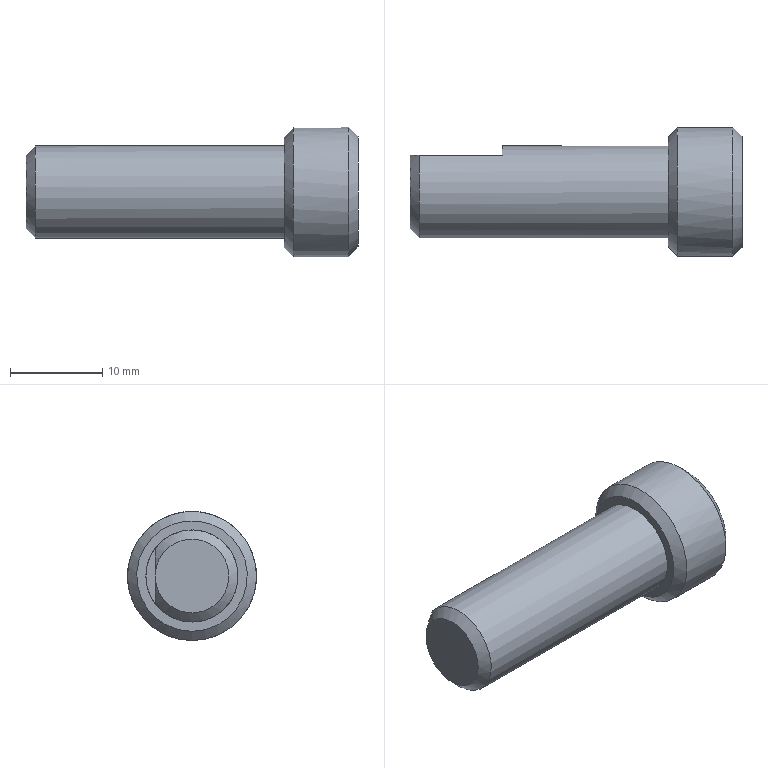Component | NX | 9_LEVER | 1 solid | 10 faces | box 36 x 14 x 14 mm | volume 3336 mm3 | plane 5 | cone 3 | cylinder 2 | commonest cylinder face diameters 10 x1 14 x1
STEP:
#1=CARTESIAN_POINT('',(0.,0.,0.));
#2=DIRECTION('',(0.,0.,1.));
#3=DIRECTION('',(1.,0.,0.));
#4=AXIS2_PLACEMENT_3D('',#1,#2,#3);
#5=CARTESIAN_POINT('',(14.,4.,75.));
#6=VERTEX_POINT('',#5);
#7=CARTESIAN_POINT('',(14.,-0.,75.));
#8=DIRECTION('',(-1.,0.,-0.));
#9=DIRECTION('',(0.,0.,-1.));
#10=AXIS2_PLACEMENT_3D('',#7,#8,#9);
#11=CIRCLE('',#10,4.);
#12=CARTESIAN_POINT('',(14.,-0.,75.));
#13=DIRECTION('',(1.,0.,0.));
#14=DIRECTION('',(0.,0.,-1.));
#15=AXIS2_PLACEMENT_3D('',#12,#13,#14);
#16=PLANE('',#15);
#17=CARTESIAN_POINT('',(4.,0.));
#18=CARTESIAN_POINT('',(4.,-6.928));
#19=CARTESIAN_POINT('',(-2.,-3.464));
#20=CARTESIAN_POINT('',(-8.,-0.));
#21=CARTESIAN_POINT('',(-2.,3.464));
#22=CARTESIAN_POINT('',(4.,6.928));
#23=CARTESIAN_POINT('',(4.,0.));
#24=(BOUNDED_CURVE()B_SPLINE_CURVE(2,(#17,#18,#19,#20,#21,#22,#23),.UNSPECIFIED.,.T.,.F.)B_SPLINE_CURVE_WITH_KNOTS((1,2,2,2,2,1),(-2.094,0.,2.094,4.189,6.283,8.378),.UNSPECIFIED.)CURVE()GEOMETRIC_REPRESENTATION_ITEM()RATIONAL_B_SPLINE_CURVE((1.,0.5,1.,0.5,1.,0.5,1.))REPRESENTATION_ITEM(''));
#25=(GEOMETRIC_REPRESENTATION_CONTEXT(2)PARAMETRIC_REPRESENTATION_CONTEXT()REPRESENTATION_CONTEXT('',''));
#26=DEFINITIONAL_REPRESENTATION('',(#24),#25);
#27=PCURVE('',#16,#26);
#28=CARTESIAN_POINT('',(15.,-0.,75.));
#29=DIRECTION('',(1.,0.,0.));
#30=DIRECTION('',(0.,0.,-1.));
#31=AXIS2_PLACEMENT_3D('',#28,#29,#30);
#32=CONICAL_SURFACE('',#31,5.,0.7854);
#33=CARTESIAN_POINT('',(12.566,-1.));
#34=DIRECTION('',(-1.,0.));
#35=VECTOR('',#34,1.);
#36=LINE('',#33,#35);
#37=(GEOMETRIC_REPRESENTATION_CONTEXT(2)PARAMETRIC_REPRESENTATION_CONTEXT()REPRESENTATION_CONTEXT('',''));
#38=DEFINITIONAL_REPRESENTATION('',(#36),#37);
#39=PCURVE('',#32,#38);
#40=SURFACE_CURVE('',#11,(#27,#39),.PCURVE_S1.);
#41=EDGE_CURVE('',#6,#6,#40,.T.);
#42=ORIENTED_EDGE('',*,*,#41,.T.);
#43=EDGE_LOOP('',(#42));
#44=FACE_BOUND('',#43,.T.);
#45=ADVANCED_FACE('',(#44),#16,.F.);
#46=CARTESIAN_POINT('',(50.,-0.,81.));
#47=VERTEX_POINT('',#46);
#48=CARTESIAN_POINT('',(50.,-0.,75.));
#49=DIRECTION('',(1.,0.,0.));
#50=DIRECTION('',(-0.,0.,1.));
#51=AXIS2_PLACEMENT_3D('',#48,#49,#50);
#52=CIRCLE('',#51,6.);
#53=CARTESIAN_POINT('',(50.,-0.,82.));
#54=DIRECTION('',(-1.,0.,-0.));
#55=DIRECTION('',(-0.,0.,1.));
#56=AXIS2_PLACEMENT_3D('',#53,#54,#55);
#57=PLANE('',#56);
#58=CARTESIAN_POINT('',(-1.,0.));
#59=CARTESIAN_POINT('',(-1.,-10.392));
#60=CARTESIAN_POINT('',(-10.,-5.196));
#61=CARTESIAN_POINT('',(-19.,-0.));
#62=CARTESIAN_POINT('',(-10.,5.196));
#63=CARTESIAN_POINT('',(-1.,10.392));
#64=CARTESIAN_POINT('',(-1.,0.));
#65=(BOUNDED_CURVE()B_SPLINE_CURVE(2,(#58,#59,#60,#61,#62,#63,#64),.UNSPECIFIED.,.T.,.F.)B_SPLINE_CURVE_WITH_KNOTS((1,2,2,2,2,1),(-2.094,0.,2.094,4.189,6.283,8.378),.UNSPECIFIED.)CURVE()GEOMETRIC_REPRESENTATION_ITEM()RATIONAL_B_SPLINE_CURVE((1.,0.5,1.,0.5,1.,0.5,1.))REPRESENTATION_ITEM(''));
#66=(GEOMETRIC_REPRESENTATION_CONTEXT(2)PARAMETRIC_REPRESENTATION_CONTEXT()REPRESENTATION_CONTEXT('',''));
#67=DEFINITIONAL_REPRESENTATION('',(#65),#66);
#68=PCURVE('',#57,#67);
#69=CARTESIAN_POINT('',(50.,-0.,75.));
#70=DIRECTION('',(-1.,0.,-0.));
#71=DIRECTION('',(-0.,0.,1.));
#72=AXIS2_PLACEMENT_3D('',#69,#70,#71);
#73=CONICAL_SURFACE('',#72,6.,0.7854);
#74=CARTESIAN_POINT('',(6.283,0.));
#75=DIRECTION('',(-1.,0.));
#76=VECTOR('',#75,1.);
#77=LINE('',#74,#76);
#78=(GEOMETRIC_REPRESENTATION_CONTEXT(2)PARAMETRIC_REPRESENTATION_CONTEXT()REPRESENTATION_CONTEXT('',''));
#79=DEFINITIONAL_REPRESENTATION('',(#77),#78);
#80=PCURVE('',#73,#79);
#81=SURFACE_CURVE('',#52,(#68,#80),.PCURVE_S1.);
#82=EDGE_CURVE('',#47,#47,#81,.T.);
#83=ORIENTED_EDGE('',*,*,#82,.T.);
#84=EDGE_LOOP('',(#83));
#85=FACE_BOUND('',#84,.T.);
#86=ADVANCED_FACE('',(#85),#57,.F.);
#87=CARTESIAN_POINT('',(24.,4.,78.));
#88=VERTEX_POINT('',#87);
#89=CARTESIAN_POINT('',(15.,4.,78.));
#90=VERTEX_POINT('',#89);
#91=CARTESIAN_POINT('',(14.,4.,78.));
#92=DIRECTION('',(-1.,0.,-0.));
#93=VECTOR('',#92,1.);
#94=LINE('',#91,#93);
#95=CARTESIAN_POINT('',(14.,-0.,75.));
#96=DIRECTION('',(1.,0.,0.));
#97=DIRECTION('',(0.,0.,-1.));
#98=AXIS2_PLACEMENT_3D('',#95,#96,#97);
#99=CYLINDRICAL_SURFACE('',#98,5.);
#100=CARTESIAN_POINT('',(2.214,0.));
#101=DIRECTION('',(0.,-1.));
#102=VECTOR('',#101,1.);
#103=LINE('',#100,#102);
#104=(GEOMETRIC_REPRESENTATION_CONTEXT(2)PARAMETRIC_REPRESENTATION_CONTEXT()REPRESENTATION_CONTEXT('',''));
#105=DEFINITIONAL_REPRESENTATION('',(#103),#104);
#106=PCURVE('',#99,#105);
#107=CARTESIAN_POINT('',(24.,4.,71.));
#108=DIRECTION('',(0.,-1.,0.));
#109=DIRECTION('',(0.,0.,1.));
#110=AXIS2_PLACEMENT_3D('',#107,#108,#109);
#111=PLANE('',#110);
#112=CARTESIAN_POINT('',(7.,10.));
#113=DIRECTION('',(-0.,1.));
#114=VECTOR('',#113,1.);
#115=LINE('',#112,#114);
#116=(GEOMETRIC_REPRESENTATION_CONTEXT(2)PARAMETRIC_REPRESENTATION_CONTEXT()REPRESENTATION_CONTEXT('',''));
#117=DEFINITIONAL_REPRESENTATION('',(#115),#116);
#118=PCURVE('',#111,#117);
#119=SURFACE_CURVE('',#94,(#106,#118),.PCURVE_S1.);
#120=EDGE_CURVE('',#88,#90,#119,.T.);
#121=ORIENTED_EDGE('',*,*,#120,.T.);
#122=CARTESIAN_POINT('',(15.,-0.,70.));
#123=VERTEX_POINT('',#122);
#124=CARTESIAN_POINT('',(15.,-0.,75.));
#125=DIRECTION('',(1.,0.,0.));
#126=DIRECTION('',(0.,0.,-1.));
#127=AXIS2_PLACEMENT_3D('',#124,#125,#126);
#128=CIRCLE('',#127,5.);
#129=CARTESIAN_POINT('',(0.,1.));
#130=DIRECTION('',(1.,0.));
#131=VECTOR('',#130,1.);
#132=LINE('',#129,#131);
#133=(GEOMETRIC_REPRESENTATION_CONTEXT(2)PARAMETRIC_REPRESENTATION_CONTEXT()REPRESENTATION_CONTEXT('',''));
#134=DEFINITIONAL_REPRESENTATION('',(#132),#133);
#135=PCURVE('',#99,#134);
#136=CARTESIAN_POINT('',(0.,0.));
#137=DIRECTION('',(1.,0.));
#138=VECTOR('',#137,1.);
#139=LINE('',#136,#138);
#140=(GEOMETRIC_REPRESENTATION_CONTEXT(2)PARAMETRIC_REPRESENTATION_CONTEXT()REPRESENTATION_CONTEXT('',''));
#141=DEFINITIONAL_REPRESENTATION('',(#139),#140);
#142=PCURVE('',#32,#141);
#143=SURFACE_CURVE('',#128,(#135,#142),.PCURVE_S1.);
#144=EDGE_CURVE('',#90,#123,#143,.T.);
#145=ORIENTED_EDGE('',*,*,#144,.T.);
#146=CARTESIAN_POINT('',(42.,-0.,70.));
#147=VERTEX_POINT('',#146);
#148=CARTESIAN_POINT('',(15.,-0.,70.));
#149=CARTESIAN_POINT('',(42.,-0.,70.));
#150=B_SPLINE_CURVE_WITH_KNOTS('',1,(#148,#149),.UNSPECIFIED.,.F.,.F.,(2,2),(1.,28.),.PIECEWISE_BEZIER_KNOTS.);
#151=CARTESIAN_POINT('',(6.283,0.));
#152=DIRECTION('',(0.,1.));
#153=VECTOR('',#152,1.);
#154=LINE('',#151,#153);
#155=(GEOMETRIC_REPRESENTATION_CONTEXT(2)PARAMETRIC_REPRESENTATION_CONTEXT()REPRESENTATION_CONTEXT('',''));
#156=DEFINITIONAL_REPRESENTATION('',(#154),#155);
#157=PCURVE('',#99,#156);
#158=CARTESIAN_POINT('',(0.,0.));
#159=DIRECTION('',(0.,1.));
#160=VECTOR('',#159,1.);
#161=LINE('',#158,#160);
#162=(GEOMETRIC_REPRESENTATION_CONTEXT(2)PARAMETRIC_REPRESENTATION_CONTEXT()REPRESENTATION_CONTEXT('',''));
#163=DEFINITIONAL_REPRESENTATION('',(#161),#162);
#164=PCURVE('',#99,#163);
#165=SEAM_CURVE('',#150,(#157,#164),.PCURVE_S1.);
#166=EDGE_CURVE('',#123,#147,#165,.T.);
#167=ORIENTED_EDGE('',*,*,#166,.T.);
#168=CARTESIAN_POINT('',(42.,-0.,75.));
#169=DIRECTION('',(1.,0.,0.));
#170=DIRECTION('',(0.,0.,-1.));
#171=AXIS2_PLACEMENT_3D('',#168,#169,#170);
#172=CIRCLE('',#171,5.);
#173=CARTESIAN_POINT('',(0.,28.));
#174=DIRECTION('',(1.,0.));
#175=VECTOR('',#174,1.);
#176=LINE('',#173,#175);
#177=(GEOMETRIC_REPRESENTATION_CONTEXT(2)PARAMETRIC_REPRESENTATION_CONTEXT()REPRESENTATION_CONTEXT('',''));
#178=DEFINITIONAL_REPRESENTATION('',(#176),#177);
#179=PCURVE('',#99,#178);
#180=CARTESIAN_POINT('',(42.,-0.,80.));
#181=DIRECTION('',(1.,0.,0.));
#182=DIRECTION('',(0.,0.,-1.));
#183=AXIS2_PLACEMENT_3D('',#180,#181,#182);
#184=PLANE('',#183);
#185=CARTESIAN_POINT('',(5.,0.));
#186=DIRECTION('',(1.,0.));
#187=AXIS2_PLACEMENT_2D('',#185,#186);
#188=CIRCLE('',#187,5.);
#189=(GEOMETRIC_REPRESENTATION_CONTEXT(2)PARAMETRIC_REPRESENTATION_CONTEXT()REPRESENTATION_CONTEXT('',''));
#190=DEFINITIONAL_REPRESENTATION('',(#188),#189);
#191=PCURVE('',#184,#190);
#192=SURFACE_CURVE('',#172,(#179,#191),.PCURVE_S1.);
#193=EDGE_CURVE('',#147,#147,#192,.T.);
#194=ORIENTED_EDGE('',*,*,#193,.F.);
#195=ORIENTED_EDGE('',*,*,#166,.F.);
#196=CARTESIAN_POINT('',(15.,4.,72.));
#197=VERTEX_POINT('',#196);
#198=CARTESIAN_POINT('',(15.,-0.,75.));
#199=DIRECTION('',(1.,0.,0.));
#200=DIRECTION('',(0.,0.,-1.));
#201=AXIS2_PLACEMENT_3D('',#198,#199,#200);
#202=CIRCLE('',#201,5.);
#203=CARTESIAN_POINT('',(-6.283,1.));
#204=DIRECTION('',(1.,0.));
#205=VECTOR('',#204,1.);
#206=LINE('',#203,#205);
#207=(GEOMETRIC_REPRESENTATION_CONTEXT(2)PARAMETRIC_REPRESENTATION_CONTEXT()REPRESENTATION_CONTEXT('',''));
#208=DEFINITIONAL_REPRESENTATION('',(#206),#207);
#209=PCURVE('',#99,#208);
#210=CARTESIAN_POINT('',(0.,0.));
#211=DIRECTION('',(1.,-0.));
#212=VECTOR('',#211,1.);
#213=LINE('',#210,#212);
#214=(GEOMETRIC_REPRESENTATION_CONTEXT(2)PARAMETRIC_REPRESENTATION_CONTEXT()REPRESENTATION_CONTEXT('',''));
#215=DEFINITIONAL_REPRESENTATION('',(#213),#214);
#216=PCURVE('',#32,#215);
#217=SURFACE_CURVE('',#202,(#209,#216),.PCURVE_S1.);
#218=EDGE_CURVE('',#123,#197,#217,.T.);
#219=ORIENTED_EDGE('',*,*,#218,.T.);
#220=CARTESIAN_POINT('',(24.,4.,72.));
#221=VERTEX_POINT('',#220);
#222=CARTESIAN_POINT('',(14.,4.,72.));
#223=DIRECTION('',(1.,0.,0.));
#224=VECTOR('',#223,1.);
#225=LINE('',#222,#224);
#226=CARTESIAN_POINT('',(0.9273,0.));
#227=DIRECTION('',(0.,1.));
#228=VECTOR('',#227,1.);
#229=LINE('',#226,#228);
#230=(GEOMETRIC_REPRESENTATION_CONTEXT(2)PARAMETRIC_REPRESENTATION_CONTEXT()REPRESENTATION_CONTEXT('',''));
#231=DEFINITIONAL_REPRESENTATION('',(#229),#230);
#232=PCURVE('',#99,#231);
#233=CARTESIAN_POINT('',(1.,10.));
#234=DIRECTION('',(0.,-1.));
#235=VECTOR('',#234,1.);
#236=LINE('',#233,#235);
#237=(GEOMETRIC_REPRESENTATION_CONTEXT(2)PARAMETRIC_REPRESENTATION_CONTEXT()REPRESENTATION_CONTEXT('',''));
#238=DEFINITIONAL_REPRESENTATION('',(#236),#237);
#239=PCURVE('',#111,#238);
#240=SURFACE_CURVE('',#225,(#232,#239),.PCURVE_S1.);
#241=EDGE_CURVE('',#197,#221,#240,.T.);
#242=ORIENTED_EDGE('',*,*,#241,.T.);
#243=CARTESIAN_POINT('',(24.,-0.,75.));
#244=DIRECTION('',(-1.,0.,0.));
#245=DIRECTION('',(0.,0.,1.));
#246=AXIS2_PLACEMENT_3D('',#243,#244,#245);
#247=CIRCLE('',#246,5.);
#248=CARTESIAN_POINT('',(3.142,10.));
#249=DIRECTION('',(-1.,0.));
#250=VECTOR('',#249,1.);
#251=LINE('',#248,#250);
#252=(GEOMETRIC_REPRESENTATION_CONTEXT(2)PARAMETRIC_REPRESENTATION_CONTEXT()REPRESENTATION_CONTEXT('',''));
#253=DEFINITIONAL_REPRESENTATION('',(#251),#252);
#254=PCURVE('',#99,#253);
#255=CARTESIAN_POINT('',(24.,-0.,75.));
#256=DIRECTION('',(-1.,0.,0.));
#257=DIRECTION('',(0.,0.,1.));
#258=AXIS2_PLACEMENT_3D('',#255,#256,#257);
#259=PLANE('',#258);
#260=CARTESIAN_POINT('',(0.,0.));
#261=DIRECTION('',(1.,0.));
#262=AXIS2_PLACEMENT_2D('',#260,#261);
#263=CIRCLE('',#262,5.);
#264=(GEOMETRIC_REPRESENTATION_CONTEXT(2)PARAMETRIC_REPRESENTATION_CONTEXT()REPRESENTATION_CONTEXT('',''));
#265=DEFINITIONAL_REPRESENTATION('',(#263),#264);
#266=PCURVE('',#259,#265);
#267=SURFACE_CURVE('',#247,(#254,#266),.PCURVE_S1.);
#268=EDGE_CURVE('',#88,#221,#267,.T.);
#269=ORIENTED_EDGE('',*,*,#268,.F.);
#270=EDGE_LOOP('',(#121,#145,#167,#194,#195,#219,#242,#269));
#271=FACE_BOUND('',#270,.T.);
#272=ADVANCED_FACE('',(#271),#99,.T.);
#273=CARTESIAN_POINT('',(42.,-0.,69.));
#274=VERTEX_POINT('',#273);
#275=CARTESIAN_POINT('',(42.,-0.,75.));
#276=DIRECTION('',(-1.,0.,-0.));
#277=DIRECTION('',(0.,0.,-1.));
#278=AXIS2_PLACEMENT_3D('',#275,#276,#277);
#279=CIRCLE('',#278,6.);
#280=CARTESIAN_POINT('',(11.,0.));
#281=CARTESIAN_POINT('',(11.,-10.392));
#282=CARTESIAN_POINT('',(2.,-5.196));
#283=CARTESIAN_POINT('',(-7.,-0.));
#284=CARTESIAN_POINT('',(2.,5.196));
#285=CARTESIAN_POINT('',(11.,10.392));
#286=CARTESIAN_POINT('',(11.,0.));
#287=(BOUNDED_CURVE()B_SPLINE_CURVE(2,(#280,#281,#282,#283,#284,#285,#286),.UNSPECIFIED.,.T.,.F.)B_SPLINE_CURVE_WITH_KNOTS((1,2,2,2,2,1),(-2.094,0.,2.094,4.189,6.283,8.378),.UNSPECIFIED.)CURVE()GEOMETRIC_REPRESENTATION_ITEM()RATIONAL_B_SPLINE_CURVE((1.,0.5,1.,0.5,1.,0.5,1.))REPRESENTATION_ITEM(''));
#288=(GEOMETRIC_REPRESENTATION_CONTEXT(2)PARAMETRIC_REPRESENTATION_CONTEXT()REPRESENTATION_CONTEXT('',''));
#289=DEFINITIONAL_REPRESENTATION('',(#287),#288);
#290=PCURVE('',#184,#289);
#291=CARTESIAN_POINT('',(43.,-0.,75.));
#292=DIRECTION('',(1.,0.,0.));
#293=DIRECTION('',(0.,0.,-1.));
#294=AXIS2_PLACEMENT_3D('',#291,#292,#293);
#295=CONICAL_SURFACE('',#294,7.,0.7854);
#296=CARTESIAN_POINT('',(6.283,-1.));
#297=DIRECTION('',(-1.,0.));
#298=VECTOR('',#297,1.);
#299=LINE('',#296,#298);
#300=(GEOMETRIC_REPRESENTATION_CONTEXT(2)PARAMETRIC_REPRESENTATION_CONTEXT()REPRESENTATION_CONTEXT('',''));
#301=DEFINITIONAL_REPRESENTATION('',(#299),#300);
#302=PCURVE('',#295,#301);
#303=SURFACE_CURVE('',#279,(#290,#302),.PCURVE_S1.);
#304=EDGE_CURVE('',#274,#274,#303,.T.);
#305=ORIENTED_EDGE('',*,*,#304,.T.);
#306=EDGE_LOOP('',(#305));
#307=FACE_BOUND('',#306,.T.);
#308=ORIENTED_EDGE('',*,*,#193,.T.);
#309=EDGE_LOOP('',(#308));
#310=FACE_BOUND('',#309,.T.);
#311=ADVANCED_FACE('',(#307,#310),#184,.F.);
#312=CARTESIAN_POINT('',(49.,-0.,82.));
#313=VERTEX_POINT('',#312);
#314=CARTESIAN_POINT('',(49.,-0.,68.));
#315=VERTEX_POINT('',#314);
#316=CARTESIAN_POINT('',(49.,-0.,75.));
#317=DIRECTION('',(-1.,0.,-0.));
#318=DIRECTION('',(-0.,0.,1.));
#319=AXIS2_PLACEMENT_3D('',#316,#317,#318);
#320=CIRCLE('',#319,7.);
#321=CARTESIAN_POINT('',(14.,-0.,75.));
#322=DIRECTION('',(1.,0.,0.));
#323=DIRECTION('',(0.,0.,-1.));
#324=AXIS2_PLACEMENT_3D('',#321,#322,#323);
#325=CYLINDRICAL_SURFACE('',#324,7.);
#326=CARTESIAN_POINT('',(3.142,35.));
#327=DIRECTION('',(-1.,0.));
#328=VECTOR('',#327,1.);
#329=LINE('',#326,#328);
#330=(GEOMETRIC_REPRESENTATION_CONTEXT(2)PARAMETRIC_REPRESENTATION_CONTEXT()REPRESENTATION_CONTEXT('',''));
#331=DEFINITIONAL_REPRESENTATION('',(#329),#330);
#332=PCURVE('',#325,#331);
#333=CARTESIAN_POINT('',(0.,1.));
#334=DIRECTION('',(1.,0.));
#335=VECTOR('',#334,1.);
#336=LINE('',#333,#335);
#337=(GEOMETRIC_REPRESENTATION_CONTEXT(2)PARAMETRIC_REPRESENTATION_CONTEXT()REPRESENTATION_CONTEXT('',''));
#338=DEFINITIONAL_REPRESENTATION('',(#336),#337);
#339=PCURVE('',#73,#338);
#340=SURFACE_CURVE('',#320,(#332,#339),.PCURVE_S1.);
#341=EDGE_CURVE('',#313,#315,#340,.T.);
#342=ORIENTED_EDGE('',*,*,#341,.T.);
#343=CARTESIAN_POINT('',(43.,-0.,68.));
#344=VERTEX_POINT('',#343);
#345=CARTESIAN_POINT('',(43.,-0.,68.));
#346=CARTESIAN_POINT('',(49.,-0.,68.));
#347=B_SPLINE_CURVE_WITH_KNOTS('',1,(#345,#346),.UNSPECIFIED.,.F.,.F.,(2,2),(29.,35.),.PIECEWISE_BEZIER_KNOTS.);
#348=CARTESIAN_POINT('',(0.,0.));
#349=DIRECTION('',(0.,1.));
#350=VECTOR('',#349,1.);
#351=LINE('',#348,#350);
#352=(GEOMETRIC_REPRESENTATION_CONTEXT(2)PARAMETRIC_REPRESENTATION_CONTEXT()REPRESENTATION_CONTEXT('',''));
#353=DEFINITIONAL_REPRESENTATION('',(#351),#352);
#354=PCURVE('',#325,#353);
#355=CARTESIAN_POINT('',(6.283,0.));
#356=DIRECTION('',(0.,1.));
#357=VECTOR('',#356,1.);
#358=LINE('',#355,#357);
#359=(GEOMETRIC_REPRESENTATION_CONTEXT(2)PARAMETRIC_REPRESENTATION_CONTEXT()REPRESENTATION_CONTEXT('',''));
#360=DEFINITIONAL_REPRESENTATION('',(#358),#359);
#361=PCURVE('',#325,#360);
#362=SEAM_CURVE('',#347,(#354,#361),.PCURVE_S1.);
#363=EDGE_CURVE('',#344,#315,#362,.T.);
#364=ORIENTED_EDGE('',*,*,#363,.F.);
#365=CARTESIAN_POINT('',(43.,-0.,75.));
#366=DIRECTION('',(1.,0.,0.));
#367=DIRECTION('',(0.,0.,-1.));
#368=AXIS2_PLACEMENT_3D('',#365,#366,#367);
#369=CIRCLE('',#368,7.);
#370=CARTESIAN_POINT('',(0.,29.));
#371=DIRECTION('',(1.,0.));
#372=VECTOR('',#371,1.);
#373=LINE('',#370,#372);
#374=(GEOMETRIC_REPRESENTATION_CONTEXT(2)PARAMETRIC_REPRESENTATION_CONTEXT()REPRESENTATION_CONTEXT('',''));
#375=DEFINITIONAL_REPRESENTATION('',(#373),#374);
#376=PCURVE('',#325,#375);
#377=CARTESIAN_POINT('',(0.,0.));
#378=DIRECTION('',(1.,0.));
#379=VECTOR('',#378,1.);
#380=LINE('',#377,#379);
#381=(GEOMETRIC_REPRESENTATION_CONTEXT(2)PARAMETRIC_REPRESENTATION_CONTEXT()REPRESENTATION_CONTEXT('',''));
#382=DEFINITIONAL_REPRESENTATION('',(#380),#381);
#383=PCURVE('',#295,#382);
#384=SURFACE_CURVE('',#369,(#376,#383),.PCURVE_S1.);
#385=EDGE_CURVE('',#344,#344,#384,.T.);
#386=ORIENTED_EDGE('',*,*,#385,.T.);
#387=ORIENTED_EDGE('',*,*,#363,.T.);
#388=CARTESIAN_POINT('',(49.,-0.,75.));
#389=DIRECTION('',(-1.,0.,-0.));
#390=DIRECTION('',(-0.,0.,1.));
#391=AXIS2_PLACEMENT_3D('',#388,#389,#390);
#392=CIRCLE('',#391,7.);
#393=CARTESIAN_POINT('',(9.425,35.));
#394=DIRECTION('',(-1.,0.));
#395=VECTOR('',#394,1.);
#396=LINE('',#393,#395);
#397=(GEOMETRIC_REPRESENTATION_CONTEXT(2)PARAMETRIC_REPRESENTATION_CONTEXT()REPRESENTATION_CONTEXT('',''));
#398=DEFINITIONAL_REPRESENTATION('',(#396),#397);
#399=PCURVE('',#325,#398);
#400=CARTESIAN_POINT('',(0.,1.));
#401=DIRECTION('',(1.,0.));
#402=VECTOR('',#401,1.);
#403=LINE('',#400,#402);
#404=(GEOMETRIC_REPRESENTATION_CONTEXT(2)PARAMETRIC_REPRESENTATION_CONTEXT()REPRESENTATION_CONTEXT('',''));
#405=DEFINITIONAL_REPRESENTATION('',(#403),#404);
#406=PCURVE('',#73,#405);
#407=SURFACE_CURVE('',#392,(#399,#406),.PCURVE_S1.);
#408=EDGE_CURVE('',#315,#313,#407,.T.);
#409=ORIENTED_EDGE('',*,*,#408,.T.);
#410=EDGE_LOOP('',(#342,#364,#386,#387,#409));
#411=FACE_BOUND('',#410,.T.);
#412=ADVANCED_FACE('',(#411),#325,.T.);
#413=ORIENTED_EDGE('',*,*,#241,.F.);
#414=CARTESIAN_POINT('',(15.,4.,72.));
#415=CARTESIAN_POINT('',(14.45,4.,72.917));
#416=CARTESIAN_POINT('',(14.,4.,73.923));
#417=CARTESIAN_POINT('',(14.,4.,75.));
#418=B_SPLINE_CURVE_WITH_KNOTS('',3,(#414,#415,#416,#417),.UNSPECIFIED.,.F.,.F.,(4,4),(0.,1.),.PIECEWISE_BEZIER_KNOTS.);
#419=CARTESIAN_POINT('',(1.,9.));
#420=CARTESIAN_POINT('',(1.917,9.55));
#421=CARTESIAN_POINT('',(2.923,10.));
#422=CARTESIAN_POINT('',(4.,10.));
#423=B_SPLINE_CURVE_WITH_KNOTS('',3,(#419,#420,#421,#422),.UNSPECIFIED.,.F.,.F.,(4,4),(0.,1.),.PIECEWISE_BEZIER_KNOTS.);
#424=(GEOMETRIC_REPRESENTATION_CONTEXT(2)PARAMETRIC_REPRESENTATION_CONTEXT()REPRESENTATION_CONTEXT('',''));
#425=DEFINITIONAL_REPRESENTATION('',(#423),#424);
#426=PCURVE('',#111,#425);
#427=CARTESIAN_POINT('',(7.21,0.));
#428=CARTESIAN_POINT('',(7.217,-0.02502));
#429=CARTESIAN_POINT('',(7.231,-0.07462));
#430=CARTESIAN_POINT('',(7.252,-0.1476));
#431=CARTESIAN_POINT('',(7.274,-0.2188));
#432=CARTESIAN_POINT('',(7.297,-0.2883));
#433=CARTESIAN_POINT('',(7.321,-0.3557));
#434=CARTESIAN_POINT('',(7.345,-0.421));
#435=CARTESIAN_POINT('',(7.371,-0.4838));
#436=CARTESIAN_POINT('',(7.397,-0.544));
#437=CARTESIAN_POINT('',(7.425,-0.6014));
#438=CARTESIAN_POINT('',(7.453,-0.6559));
#439=CARTESIAN_POINT('',(7.482,-0.7071));
#440=CARTESIAN_POINT('',(7.512,-0.7549));
#441=CARTESIAN_POINT('',(7.543,-0.7991));
#442=CARTESIAN_POINT('',(7.575,-0.8394));
#443=CARTESIAN_POINT('',(7.607,-0.8758));
#444=CARTESIAN_POINT('',(7.641,-0.9079));
#445=CARTESIAN_POINT('',(7.675,-0.9356));
#446=CARTESIAN_POINT('',(7.71,-0.9586));
#447=CARTESIAN_POINT('',(7.745,-0.9769));
#448=CARTESIAN_POINT('',(7.781,-0.9901));
#449=CARTESIAN_POINT('',(7.817,-0.9982));
#450=CARTESIAN_POINT('',(7.842,-1.));
#451=CARTESIAN_POINT('',(7.854,-1.));
#452=B_SPLINE_CURVE_WITH_KNOTS('',3,(#427,#428,#429,#430,#431,#432,#433,#434,#435,#436,#437,#438,#439,#440,#441,#442,#443,#444,#445,#446,#447,#448,#449,#450,#451),.UNSPECIFIED.,.F.,.F.,(4,1,1,1,1,1,1,1,1,1,1,1,1,1,1,1,1,1,1,1,1,1,4),(0.,0.04545,0.09091,0.1364,0.1818,0.2273,0.2727,0.3182,0.3636,0.4091,0.4545,0.5,0.5455,0.5909,0.6364,0.6818,0.7273,0.7727,0.8182,0.8636,0.9091,0.9545,1.),.QUASI_UNIFORM_KNOTS.);
#453=(GEOMETRIC_REPRESENTATION_CONTEXT(2)PARAMETRIC_REPRESENTATION_CONTEXT()REPRESENTATION_CONTEXT('',''));
#454=DEFINITIONAL_REPRESENTATION('',(#452),#453);
#455=PCURVE('',#32,#454);
#456=SURFACE_CURVE('',#418,(#426,#455),.PCURVE_S1.);
#457=EDGE_CURVE('',#197,#6,#456,.T.);
#458=ORIENTED_EDGE('',*,*,#457,.T.);
#459=CARTESIAN_POINT('',(14.,4.,75.));
#460=CARTESIAN_POINT('',(14.,4.,75.485));
#461=CARTESIAN_POINT('',(14.094,4.,75.974));
#462=CARTESIAN_POINT('',(14.249,4.,76.433));
#463=CARTESIAN_POINT('',(14.434,4.,76.982));
#464=CARTESIAN_POINT('',(14.702,4.,77.503));
#465=CARTESIAN_POINT('',(15.,4.,78.));
#466=B_SPLINE_CURVE_WITH_KNOTS('',3,(#459,#460,#461,#462,#463,#464,#465),.UNSPECIFIED.,.F.,.F.,(4,3,4),(0.,0.4568,1.),.UNSPECIFIED.);
#467=CARTESIAN_POINT('',(4.,10.));
#468=CARTESIAN_POINT('',(4.485,10.));
#469=CARTESIAN_POINT('',(4.974,9.906));
#470=CARTESIAN_POINT('',(5.433,9.751));
#471=CARTESIAN_POINT('',(5.982,9.566));
#472=CARTESIAN_POINT('',(6.503,9.298));
#473=CARTESIAN_POINT('',(7.,9.));
#474=B_SPLINE_CURVE_WITH_KNOTS('',3,(#467,#468,#469,#470,#471,#472,#473),.UNSPECIFIED.,.F.,.F.,(4,3,4),(0.,0.4568,1.),.UNSPECIFIED.);
#475=(GEOMETRIC_REPRESENTATION_CONTEXT(2)PARAMETRIC_REPRESENTATION_CONTEXT()REPRESENTATION_CONTEXT('',''));
#476=DEFINITIONAL_REPRESENTATION('',(#474),#475);
#477=PCURVE('',#111,#476);
#478=CARTESIAN_POINT('',(1.571,-1.));
#479=CARTESIAN_POINT('',(1.583,-1.));
#480=CARTESIAN_POINT('',(1.607,-0.9982));
#481=CARTESIAN_POINT('',(1.643,-0.9902));
#482=CARTESIAN_POINT('',(1.679,-0.977));
#483=CARTESIAN_POINT('',(1.715,-0.9587));
#484=CARTESIAN_POINT('',(1.75,-0.9355));
#485=CARTESIAN_POINT('',(1.784,-0.9077));
#486=CARTESIAN_POINT('',(1.818,-0.8754));
#487=CARTESIAN_POINT('',(1.851,-0.8388));
#488=CARTESIAN_POINT('',(1.883,-0.7982));
#489=CARTESIAN_POINT('',(1.913,-0.7539));
#490=CARTESIAN_POINT('',(1.944,-0.7058));
#491=CARTESIAN_POINT('',(1.973,-0.6544));
#492=CARTESIAN_POINT('',(2.001,-0.5999));
#493=CARTESIAN_POINT('',(2.028,-0.5425));
#494=CARTESIAN_POINT('',(2.055,-0.4823));
#495=CARTESIAN_POINT('',(2.08,-0.4196));
#496=CARTESIAN_POINT('',(2.105,-0.3545));
#497=CARTESIAN_POINT('',(2.128,-0.2873));
#498=CARTESIAN_POINT('',(2.151,-0.2181));
#499=CARTESIAN_POINT('',(2.173,-0.147));
#500=CARTESIAN_POINT('',(2.194,-0.07436));
#501=CARTESIAN_POINT('',(2.208,-0.02493));
#502=CARTESIAN_POINT('',(2.214,0.));
#503=B_SPLINE_CURVE_WITH_KNOTS('',3,(#478,#479,#480,#481,#482,#483,#484,#485,#486,#487,#488,#489,#490,#491,#492,#493,#494,#495,#496,#497,#498,#499,#500,#501,#502),.UNSPECIFIED.,.F.,.F.,(4,1,1,1,1,1,1,1,1,1,1,1,1,1,1,1,1,1,1,1,1,1,4),(0.,0.04545,0.09091,0.1364,0.1818,0.2273,0.2727,0.3182,0.3636,0.4091,0.4545,0.5,0.5455,0.5909,0.6364,0.6818,0.7273,0.7727,0.8182,0.8636,0.9091,0.9545,1.),.QUASI_UNIFORM_KNOTS.);
#504=(GEOMETRIC_REPRESENTATION_CONTEXT(2)PARAMETRIC_REPRESENTATION_CONTEXT()REPRESENTATION_CONTEXT('',''));
#505=DEFINITIONAL_REPRESENTATION('',(#503),#504);
#506=PCURVE('',#32,#505);
#507=SURFACE_CURVE('',#466,(#477,#506),.PCURVE_S1.);
#508=EDGE_CURVE('',#6,#90,#507,.T.);
#509=ORIENTED_EDGE('',*,*,#508,.T.);
#510=ORIENTED_EDGE('',*,*,#120,.F.);
#511=CARTESIAN_POINT('',(24.,4.,71.));
#512=DIRECTION('',(0.,-0.,-1.));
#513=VECTOR('',#512,1.);
#514=LINE('',#511,#513);
#515=CARTESIAN_POINT('',(0.,0.));
#516=DIRECTION('',(-1.,0.));
#517=VECTOR('',#516,1.);
#518=LINE('',#515,#517);
#519=(GEOMETRIC_REPRESENTATION_CONTEXT(2)PARAMETRIC_REPRESENTATION_CONTEXT()REPRESENTATION_CONTEXT('',''));
#520=DEFINITIONAL_REPRESENTATION('',(#518),#519);
#521=PCURVE('',#111,#520);
#522=CARTESIAN_POINT('',(-4.,4.));
#523=DIRECTION('',(-1.,-0.));
#524=VECTOR('',#523,1.);
#525=LINE('',#522,#524);
#526=(GEOMETRIC_REPRESENTATION_CONTEXT(2)PARAMETRIC_REPRESENTATION_CONTEXT()REPRESENTATION_CONTEXT('',''));
#527=DEFINITIONAL_REPRESENTATION('',(#525),#526);
#528=PCURVE('',#259,#527);
#529=SURFACE_CURVE('',#514,(#521,#528),.PCURVE_S1.);
#530=EDGE_CURVE('',#88,#221,#529,.T.);
#531=ORIENTED_EDGE('',*,*,#530,.T.);
#532=EDGE_LOOP('',(#413,#458,#509,#510,#531));
#533=FACE_BOUND('',#532,.T.);
#534=ADVANCED_FACE('',(#533),#111,.F.);
#535=ORIENTED_EDGE('',*,*,#268,.T.);
#536=ORIENTED_EDGE('',*,*,#530,.F.);
#537=EDGE_LOOP('',(#535,#536));
#538=FACE_BOUND('',#537,.T.);
#539=ADVANCED_FACE('',(#538),#259,.T.);
#540=ORIENTED_EDGE('',*,*,#341,.F.);
#541=CARTESIAN_POINT('',(50.,-0.,81.));
#542=CARTESIAN_POINT('',(49.,-0.,82.));
#543=B_SPLINE_CURVE_WITH_KNOTS('',1,(#541,#542),.UNSPECIFIED.,.F.,.F.,(2,2),(0.,1.414),.PIECEWISE_BEZIER_KNOTS.);
#544=CARTESIAN_POINT('',(0.,0.));
#545=DIRECTION('',(0.,1.));
#546=VECTOR('',#545,1.);
#547=LINE('',#544,#546);
#548=(GEOMETRIC_REPRESENTATION_CONTEXT(2)PARAMETRIC_REPRESENTATION_CONTEXT()REPRESENTATION_CONTEXT('',''));
#549=DEFINITIONAL_REPRESENTATION('',(#547),#548);
#550=PCURVE('',#73,#549);
#551=CARTESIAN_POINT('',(6.283,0.));
#552=DIRECTION('',(0.,1.));
#553=VECTOR('',#552,1.);
#554=LINE('',#551,#553);
#555=(GEOMETRIC_REPRESENTATION_CONTEXT(2)PARAMETRIC_REPRESENTATION_CONTEXT()REPRESENTATION_CONTEXT('',''));
#556=DEFINITIONAL_REPRESENTATION('',(#554),#555);
#557=PCURVE('',#73,#556);
#558=SEAM_CURVE('',#543,(#550,#557),.PCURVE_S1.);
#559=EDGE_CURVE('',#47,#313,#558,.T.);
#560=ORIENTED_EDGE('',*,*,#559,.F.);
#561=ORIENTED_EDGE('',*,*,#82,.F.);
#562=ORIENTED_EDGE('',*,*,#559,.T.);
#563=ORIENTED_EDGE('',*,*,#408,.F.);
#564=EDGE_LOOP('',(#540,#560,#561,#562,#563));
#565=FACE_BOUND('',#564,.T.);
#566=ADVANCED_FACE('',(#565),#73,.T.);
#567=ORIENTED_EDGE('',*,*,#304,.F.);
#568=CARTESIAN_POINT('',(42.,-0.,69.));
#569=CARTESIAN_POINT('',(43.,-0.,68.));
#570=B_SPLINE_CURVE_WITH_KNOTS('',1,(#568,#569),.UNSPECIFIED.,.F.,.F.,(2,2),(-1.414,0.),.PIECEWISE_BEZIER_KNOTS.);
#571=CARTESIAN_POINT('',(6.283,0.));
#572=DIRECTION('',(0.,1.));
#573=VECTOR('',#572,1.);
#574=LINE('',#571,#573);
#575=(GEOMETRIC_REPRESENTATION_CONTEXT(2)PARAMETRIC_REPRESENTATION_CONTEXT()REPRESENTATION_CONTEXT('',''));
#576=DEFINITIONAL_REPRESENTATION('',(#574),#575);
#577=PCURVE('',#295,#576);
#578=CARTESIAN_POINT('',(0.,0.));
#579=DIRECTION('',(0.,1.));
#580=VECTOR('',#579,1.);
#581=LINE('',#578,#580);
#582=(GEOMETRIC_REPRESENTATION_CONTEXT(2)PARAMETRIC_REPRESENTATION_CONTEXT()REPRESENTATION_CONTEXT('',''));
#583=DEFINITIONAL_REPRESENTATION('',(#581),#582);
#584=PCURVE('',#295,#583);
#585=SEAM_CURVE('',#570,(#577,#584),.PCURVE_S1.);
#586=EDGE_CURVE('',#274,#344,#585,.T.);
#587=ORIENTED_EDGE('',*,*,#586,.T.);
#588=ORIENTED_EDGE('',*,*,#385,.F.);
#589=ORIENTED_EDGE('',*,*,#586,.F.);
#590=EDGE_LOOP('',(#567,#587,#588,#589));
#591=FACE_BOUND('',#590,.T.);
#592=ADVANCED_FACE('',(#591),#295,.T.);
#593=ORIENTED_EDGE('',*,*,#508,.F.);
#594=ORIENTED_EDGE('',*,*,#41,.F.);
#595=ORIENTED_EDGE('',*,*,#457,.F.);
#596=ORIENTED_EDGE('',*,*,#218,.F.);
#597=ORIENTED_EDGE('',*,*,#144,.F.);
#598=EDGE_LOOP('',(#593,#594,#595,#596,#597));
#599=FACE_BOUND('',#598,.T.);
#600=ADVANCED_FACE('',(#599),#32,.T.);
#601=CLOSED_SHELL('',(#45,#86,#272,#311,#412,#534,#539,#566,#592,#600));
#602=MANIFOLD_SOLID_BREP('',#601);
#603=(LENGTH_UNIT()NAMED_UNIT(*)SI_UNIT(.MILLI.,.METRE.));
#604=UNCERTAINTY_MEASURE_WITH_UNIT(LENGTH_MEASURE(0.0001),#603,'','');
#605=(NAMED_UNIT(*)PLANE_ANGLE_UNIT()SI_UNIT($,.RADIAN.));
#606=(NAMED_UNIT(*)SI_UNIT($,.STERADIAN.)SOLID_ANGLE_UNIT());
#607=(GEOMETRIC_REPRESENTATION_CONTEXT(3)GLOBAL_UNCERTAINTY_ASSIGNED_CONTEXT((#604))GLOBAL_UNIT_ASSIGNED_CONTEXT((#603,#605,#606))REPRESENTATION_CONTEXT('',''));
#608=ADVANCED_BREP_SHAPE_REPRESENTATION('',(#4,#602),#607);